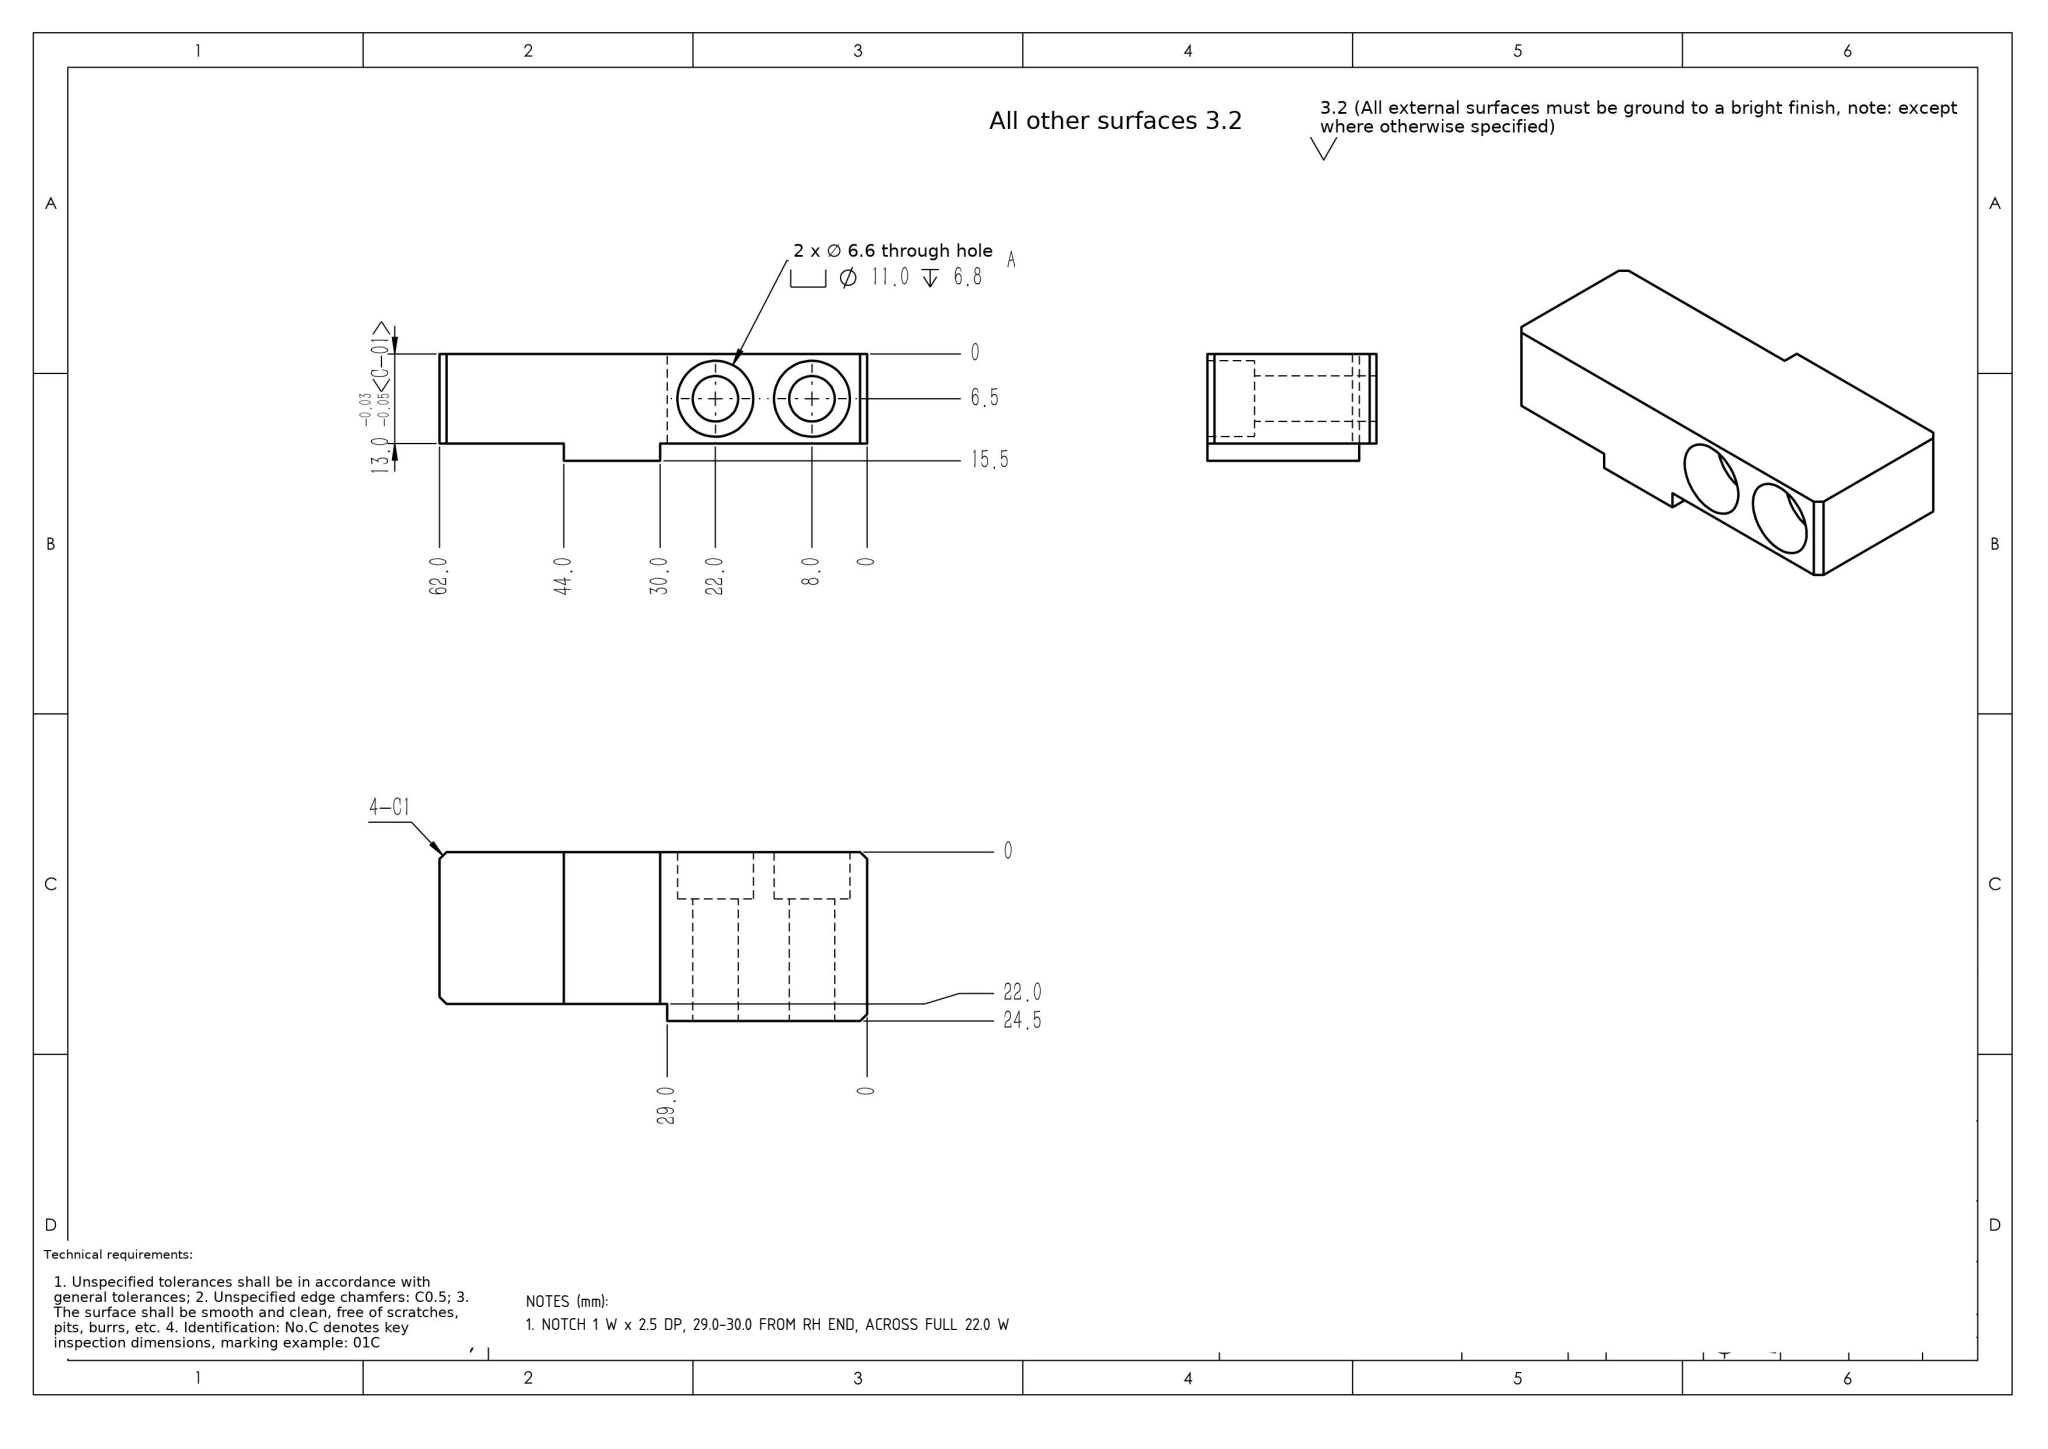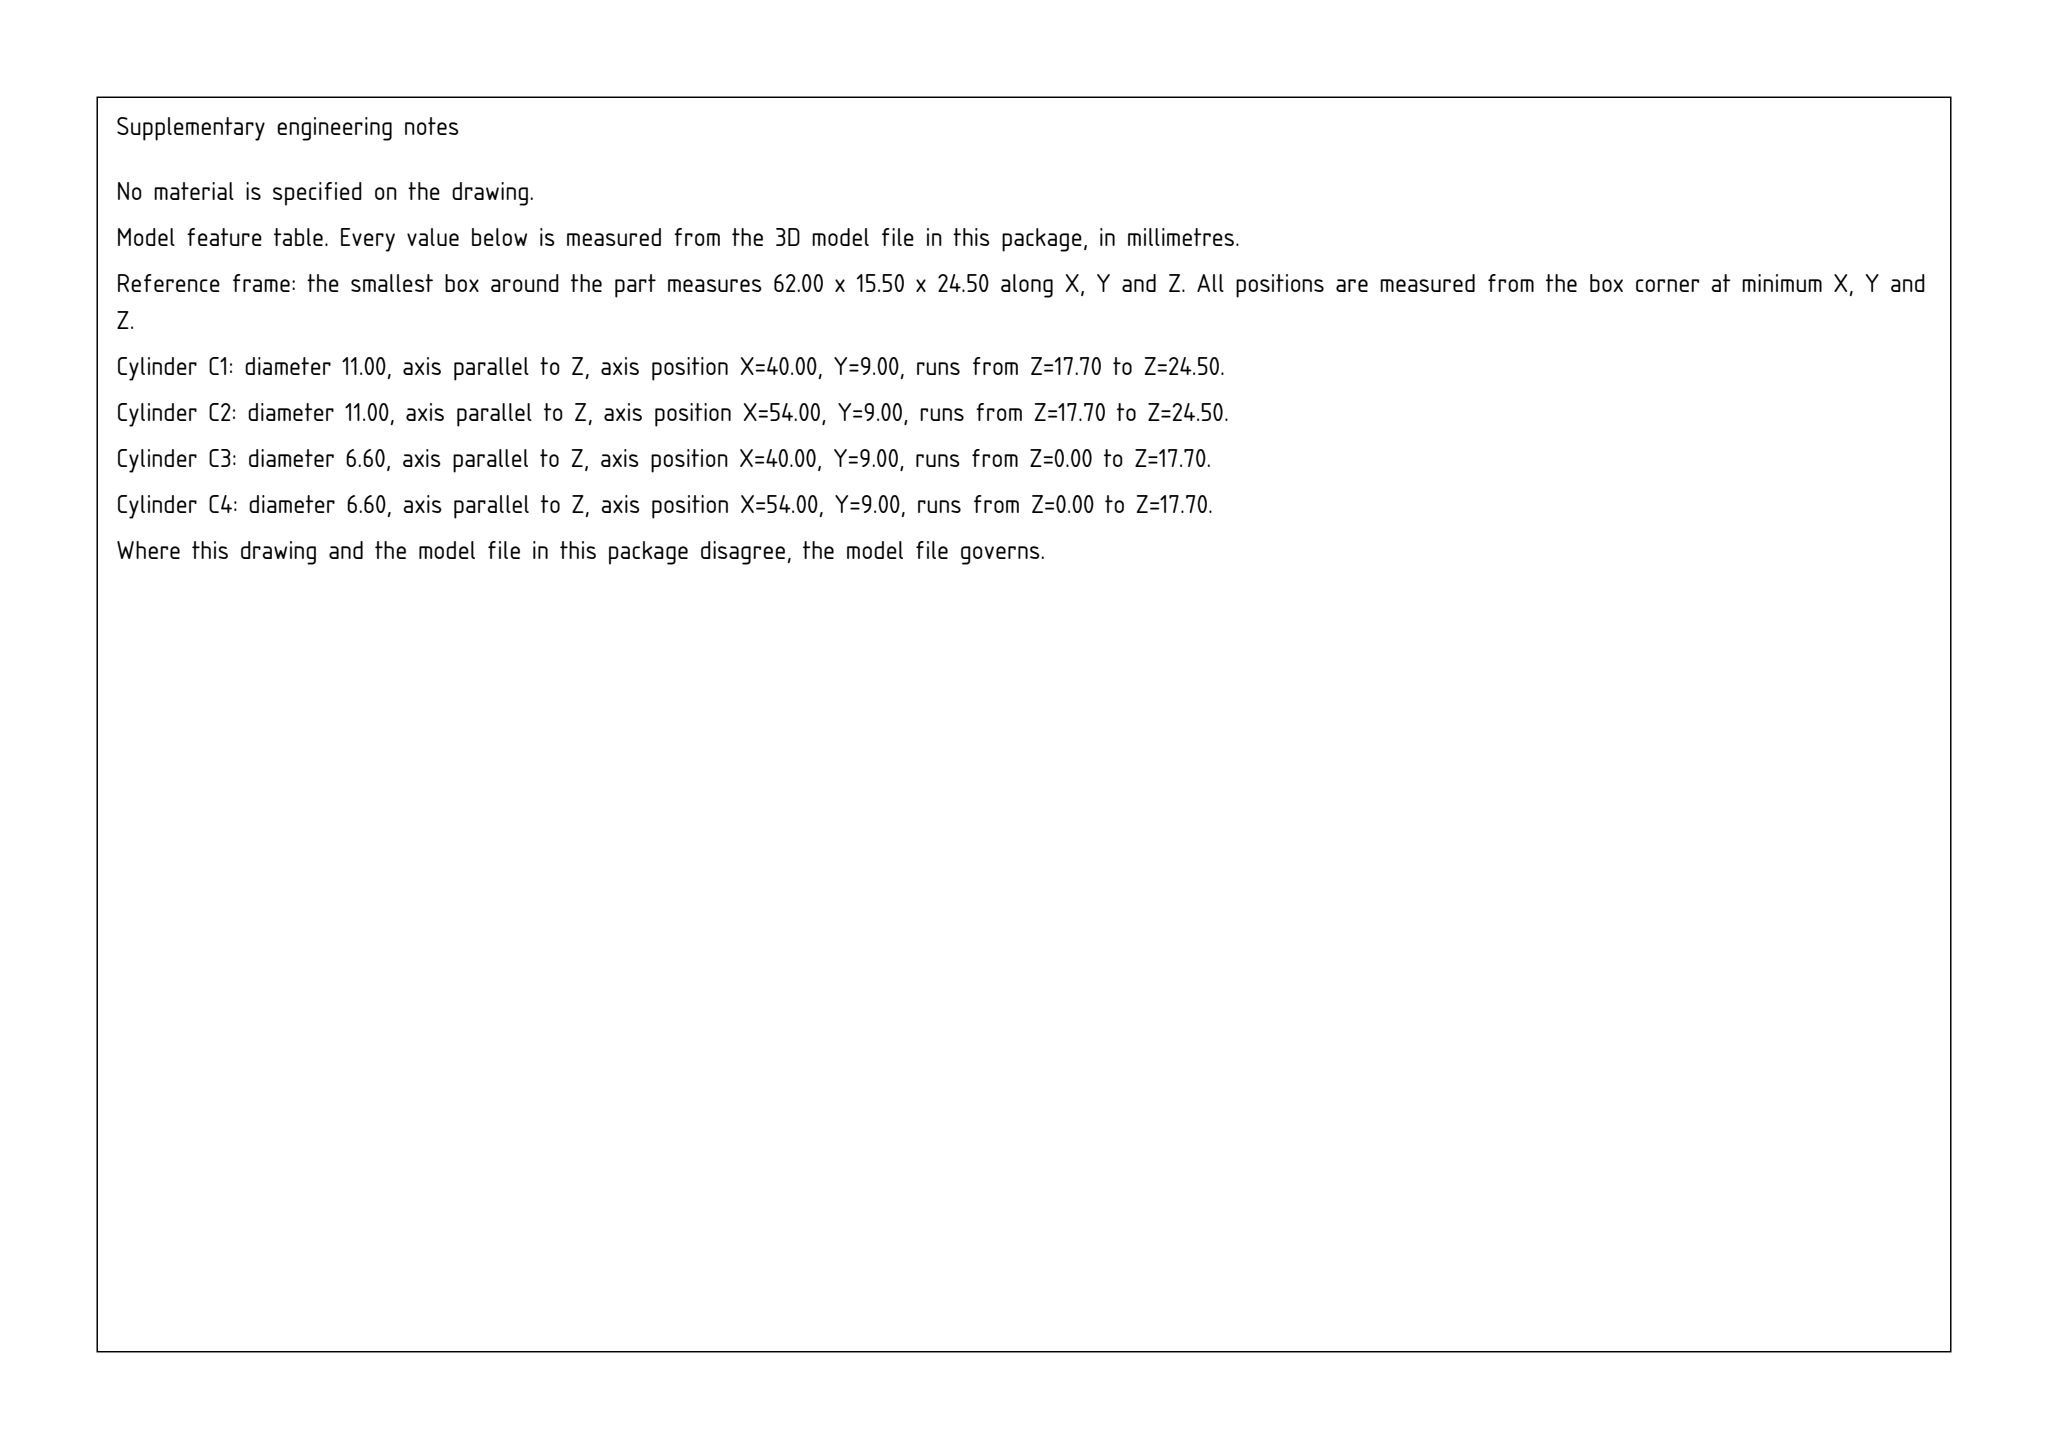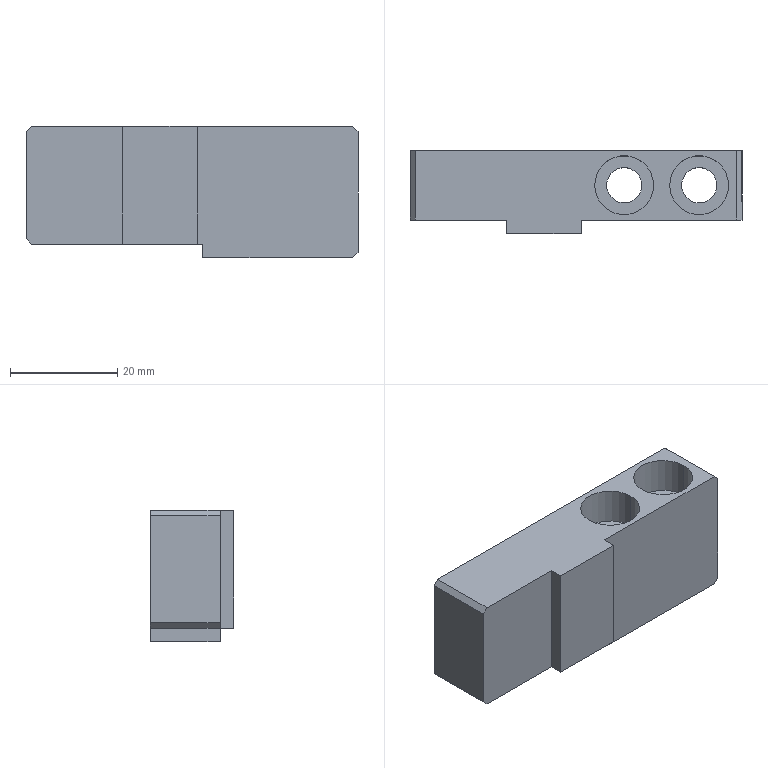Part | SolidWorks | mm | 1 solid | 26 faces | box 62 x 15.5 x 24.5 mm | volume 16915 mm3 | plane 18 | cylinder 8 | commonest cylinder face diameters 11 x4 6.6 x4
Drawing notes:
NOTCH 1 W x 2.5 DP, 29.0-30.0 FROM RH END, ACROSS FULL 22.0 W | from the solid: x-planes 32.0 & 33.0 (=29.0/30.0 from x=62 datum); 2nd y=2.5 face gives 2.5 dp; notch spans z=2.5-24.5 (22.0) as z=0-2.5 ledge ends at x=33
build123d program:
from build123d import *

# Parameters (mm, degrees)
SKETCH1_W                                          = 62
SKETCH1_H                                          = 13
BOSS_EXTRUDE1_DEPTH                                = 24.5
SKETCH2_W                                          = 33
SKETCH2_H                                          = 2.5
CUT_EXTRUDE1_DEPTH                                 = 42.596
HOLE_SIZE_ACCORDING_TO_SLOTTED_PAN_HEA_D           = 6.6
HOLE_SIZE_ACCORDING_TO_SLOTTED_PAN_HEA_CBORE_D     = 11
HOLE_SIZE_ACCORDING_TO_SLOTTED_PAN_HEA_CBORE_DEPTH = 6.8
SKETCH5_W                                          = 32
SKETCH5_H                                          = 2
BOSS_EXTRUDE2_DEPTH                                = 22
SKETCH6_W                                          = 18
SKETCH6_H                                          = 2
CUT_EXTRUDE2_DEPTH                                 = 41.417
CHAMFER1_SIZE                                      = 1
SKETCH7_W                                          = 14
SKETCH7_H                                          = 22
BOSS_EXTRUDE3_DEPTH                                = 0.5


with BuildPart() as part:
    # Sketch1 → Boss-Extrude1 (new body)
    with BuildSketch(Plane.XY):
        Rectangle(SKETCH1_W, SKETCH1_H)
    extrude(amount=BOSS_EXTRUDE1_DEPTH)

    # Sketch2 → Cut-Extrude1 (cut, through all)
    with BuildSketch(Plane(origin=(0, 6.5, 0), x_dir=(1, 0, 0), z_dir=(0, 1, 0))):
        with Locations((-14.5, -1.25)):
            Rectangle(SKETCH2_W, SKETCH2_H)
    extrude(amount=-CUT_EXTRUDE1_DEPTH, mode=Mode.SUBTRACT)

    # Hole Size _According to_ Slotted Pan Hea (through all)
    with Locations(Plane.XY.offset(24.5)):
        with Locations((9, 0), (23, 0)):
            CounterBoreHole(HOLE_SIZE_ACCORDING_TO_SLOTTED_PAN_HEA_D / 2, HOLE_SIZE_ACCORDING_TO_SLOTTED_PAN_HEA_CBORE_D / 2, HOLE_SIZE_ACCORDING_TO_SLOTTED_PAN_HEA_CBORE_DEPTH)

    # Sketch5 → Boss-Extrude2 (add)
    with BuildSketch(Plane.XY.offset(24.5)):
        with Locations((-15, -7.5)):
            Rectangle(SKETCH5_W, SKETCH5_H)
    extrude(amount=-BOSS_EXTRUDE2_DEPTH)

    # Sketch6 → Cut-Extrude2 (cut, through all)
    with BuildSketch(Plane.XY.offset(24.5)):
        with Locations((-22, -7.5)):
            Rectangle(SKETCH6_W, SKETCH6_H)
    extrude(amount=-CUT_EXTRUDE2_DEPTH, mode=Mode.SUBTRACT)

    # Chamfer1
    chamfer1_edges = [part.edges().sort_by_distance(p)[0] for p in [
        (-31, 0, 24.5),
        (31, 0, 24.5),
        (-31, 0, 2.5),
        (31, 0, 0),
    ]]
    chamfer(chamfer1_edges, length=CHAMFER1_SIZE)

    # Sketch7 → Boss-Extrude3 (add)
    with BuildSketch(Plane.XZ.offset(8.5)):
        with Locations((-6, 13.5)):
            Rectangle(SKETCH7_W, SKETCH7_H)
    extrude(amount=BOSS_EXTRUDE3_DEPTH)


solid = part.part
STEP:
#1=CARTESIAN_POINT('',(3.5,0.,17.7));
#2=VERTEX_POINT('',#1);
#3=CARTESIAN_POINT('',(14.5,0.,17.7));
#4=VERTEX_POINT('',#3);
#5=CARTESIAN_POINT('',(9.,0.,17.7));
#6=DIRECTION('',(0.,0.,1.));
#7=DIRECTION('',(1.,0.,0.));
#8=AXIS2_PLACEMENT_3D('',#5,#6,#7);
#9=CIRCLE('',#8,5.5);
#10=EDGE_CURVE('',#2,#4,#9,.T.);
#11=ORIENTED_EDGE('',*,*,#10,.F.);
#12=CARTESIAN_POINT('',(3.5,0.,24.5));
#13=VERTEX_POINT('',#12);
#14=CARTESIAN_POINT('',(3.5,0.,24.5));
#15=DIRECTION('',(0.,0.,1.));
#16=VECTOR('',#15,1000.);
#17=LINE('',#14,#16);
#18=EDGE_CURVE('',#2,#13,#17,.T.);
#19=ORIENTED_EDGE('',*,*,#18,.T.);
#20=CARTESIAN_POINT('',(14.5,0.,24.5));
#21=VERTEX_POINT('',#20);
#22=CARTESIAN_POINT('',(9.,0.,24.5));
#23=DIRECTION('',(0.,0.,1.));
#24=DIRECTION('',(1.,0.,0.));
#25=AXIS2_PLACEMENT_3D('',#22,#23,#24);
#26=CIRCLE('',#25,5.5);
#27=EDGE_CURVE('',#13,#21,#26,.T.);
#28=ORIENTED_EDGE('',*,*,#27,.T.);
#29=CARTESIAN_POINT('',(14.5,0.,24.5));
#30=DIRECTION('',(0.,0.,1.));
#31=VECTOR('',#30,1000.);
#32=LINE('',#29,#31);
#33=EDGE_CURVE('',#4,#21,#32,.T.);
#34=ORIENTED_EDGE('',*,*,#33,.F.);
#35=EDGE_LOOP('',(#11,#19,#28,#34));
#36=FACE_OUTER_BOUND('',#35,.T.);
#37=CARTESIAN_POINT('',(9.,0.,24.5));
#38=DIRECTION('',(0.,0.,1.));
#39=DIRECTION('',(1.,0.,0.));
#40=AXIS2_PLACEMENT_3D('',#37,#38,#39);
#41=CYLINDRICAL_SURFACE('',#40,5.5);
#42=ADVANCED_FACE('',(#36),#41,.F.);
#43=CARTESIAN_POINT('',(5.7,0.,0.));
#44=VERTEX_POINT('',#43);
#45=CARTESIAN_POINT('',(12.3,0.,0.));
#46=VERTEX_POINT('',#45);
#47=CARTESIAN_POINT('',(9.,0.,0.));
#48=DIRECTION('',(0.,0.,1.));
#49=DIRECTION('',(1.,0.,0.));
#50=AXIS2_PLACEMENT_3D('',#47,#48,#49);
#51=CIRCLE('',#50,3.3);
#52=EDGE_CURVE('',#44,#46,#51,.T.);
#53=ORIENTED_EDGE('',*,*,#52,.F.);
#54=CARTESIAN_POINT('',(5.7,0.,17.7));
#55=VERTEX_POINT('',#54);
#56=CARTESIAN_POINT('',(5.7,0.,24.5));
#57=DIRECTION('',(0.,0.,1.));
#58=VECTOR('',#57,1000.);
#59=LINE('',#56,#58);
#60=EDGE_CURVE('',#44,#55,#59,.T.);
#61=ORIENTED_EDGE('',*,*,#60,.T.);
#62=CARTESIAN_POINT('',(12.3,0.,17.7));
#63=VERTEX_POINT('',#62);
#64=CARTESIAN_POINT('',(9.,0.,17.7));
#65=DIRECTION('',(0.,0.,1.));
#66=DIRECTION('',(1.,0.,0.));
#67=AXIS2_PLACEMENT_3D('',#64,#65,#66);
#68=CIRCLE('',#67,3.3);
#69=EDGE_CURVE('',#55,#63,#68,.T.);
#70=ORIENTED_EDGE('',*,*,#69,.T.);
#71=CARTESIAN_POINT('',(12.3,0.,24.5));
#72=DIRECTION('',(0.,0.,1.));
#73=VECTOR('',#72,1000.);
#74=LINE('',#71,#73);
#75=EDGE_CURVE('',#46,#63,#74,.T.);
#76=ORIENTED_EDGE('',*,*,#75,.F.);
#77=EDGE_LOOP('',(#53,#61,#70,#76));
#78=FACE_OUTER_BOUND('',#77,.T.);
#79=CARTESIAN_POINT('',(9.,0.,24.5));
#80=DIRECTION('',(0.,0.,1.));
#81=DIRECTION('',(1.,0.,0.));
#82=AXIS2_PLACEMENT_3D('',#79,#80,#81);
#83=CYLINDRICAL_SURFACE('',#82,3.3);
#84=ADVANCED_FACE('',(#78),#83,.F.);
#85=CARTESIAN_POINT('',(17.5,0.,17.7));
#86=VERTEX_POINT('',#85);
#87=CARTESIAN_POINT('',(28.5,0.,17.7));
#88=VERTEX_POINT('',#87);
#89=CARTESIAN_POINT('',(23.,0.,17.7));
#90=DIRECTION('',(0.,0.,1.));
#91=DIRECTION('',(1.,0.,0.));
#92=AXIS2_PLACEMENT_3D('',#89,#90,#91);
#93=CIRCLE('',#92,5.5);
#94=EDGE_CURVE('',#86,#88,#93,.T.);
#95=ORIENTED_EDGE('',*,*,#94,.F.);
#96=CARTESIAN_POINT('',(17.5,0.,24.5));
#97=VERTEX_POINT('',#96);
#98=CARTESIAN_POINT('',(17.5,0.,24.5));
#99=DIRECTION('',(0.,0.,1.));
#100=VECTOR('',#99,1000.);
#101=LINE('',#98,#100);
#102=EDGE_CURVE('',#86,#97,#101,.T.);
#103=ORIENTED_EDGE('',*,*,#102,.T.);
#104=CARTESIAN_POINT('',(28.5,0.,24.5));
#105=VERTEX_POINT('',#104);
#106=CARTESIAN_POINT('',(23.,0.,24.5));
#107=DIRECTION('',(0.,0.,1.));
#108=DIRECTION('',(1.,0.,0.));
#109=AXIS2_PLACEMENT_3D('',#106,#107,#108);
#110=CIRCLE('',#109,5.5);
#111=EDGE_CURVE('',#97,#105,#110,.T.);
#112=ORIENTED_EDGE('',*,*,#111,.T.);
#113=CARTESIAN_POINT('',(28.5,0.,24.5));
#114=DIRECTION('',(0.,0.,1.));
#115=VECTOR('',#114,1000.);
#116=LINE('',#113,#115);
#117=EDGE_CURVE('',#88,#105,#116,.T.);
#118=ORIENTED_EDGE('',*,*,#117,.F.);
#119=EDGE_LOOP('',(#95,#103,#112,#118));
#120=FACE_OUTER_BOUND('',#119,.T.);
#121=CARTESIAN_POINT('',(23.,0.,24.5));
#122=DIRECTION('',(0.,0.,1.));
#123=DIRECTION('',(1.,0.,0.));
#124=AXIS2_PLACEMENT_3D('',#121,#122,#123);
#125=CYLINDRICAL_SURFACE('',#124,5.5);
#126=ADVANCED_FACE('',(#120),#125,.F.);
#127=CARTESIAN_POINT('',(19.7,0.,0.));
#128=VERTEX_POINT('',#127);
#129=CARTESIAN_POINT('',(26.3,0.,0.));
#130=VERTEX_POINT('',#129);
#131=CARTESIAN_POINT('',(23.,0.,0.));
#132=DIRECTION('',(0.,0.,1.));
#133=DIRECTION('',(1.,0.,0.));
#134=AXIS2_PLACEMENT_3D('',#131,#132,#133);
#135=CIRCLE('',#134,3.3);
#136=EDGE_CURVE('',#128,#130,#135,.T.);
#137=ORIENTED_EDGE('',*,*,#136,.F.);
#138=CARTESIAN_POINT('',(19.7,0.,17.7));
#139=VERTEX_POINT('',#138);
#140=CARTESIAN_POINT('',(19.7,0.,24.5));
#141=DIRECTION('',(0.,0.,1.));
#142=VECTOR('',#141,1000.);
#143=LINE('',#140,#142);
#144=EDGE_CURVE('',#128,#139,#143,.T.);
#145=ORIENTED_EDGE('',*,*,#144,.T.);
#146=CARTESIAN_POINT('',(26.3,0.,17.7));
#147=VERTEX_POINT('',#146);
#148=CARTESIAN_POINT('',(23.,0.,17.7));
#149=DIRECTION('',(0.,0.,1.));
#150=DIRECTION('',(1.,0.,0.));
#151=AXIS2_PLACEMENT_3D('',#148,#149,#150);
#152=CIRCLE('',#151,3.3);
#153=EDGE_CURVE('',#139,#147,#152,.T.);
#154=ORIENTED_EDGE('',*,*,#153,.T.);
#155=CARTESIAN_POINT('',(26.3,0.,24.5));
#156=DIRECTION('',(0.,0.,1.));
#157=VECTOR('',#156,1000.);
#158=LINE('',#155,#157);
#159=EDGE_CURVE('',#130,#147,#158,.T.);
#160=ORIENTED_EDGE('',*,*,#159,.F.);
#161=EDGE_LOOP('',(#137,#145,#154,#160));
#162=FACE_OUTER_BOUND('',#161,.T.);
#163=CARTESIAN_POINT('',(23.,0.,24.5));
#164=DIRECTION('',(0.,0.,1.));
#165=DIRECTION('',(1.,0.,0.));
#166=AXIS2_PLACEMENT_3D('',#163,#164,#165);
#167=CYLINDRICAL_SURFACE('',#166,3.3);
#168=ADVANCED_FACE('',(#162),#167,.F.);
#169=CARTESIAN_POINT('',(2.,-6.5,0.));
#170=VERTEX_POINT('',#169);
#171=CARTESIAN_POINT('',(30.,-6.5,-0.));
#172=VERTEX_POINT('',#171);
#173=CARTESIAN_POINT('',(-31.,-6.5,0.));
#174=DIRECTION('',(1.,0.,0.));
#175=VECTOR('',#174,1000.);
#176=LINE('',#173,#175);
#177=EDGE_CURVE('',#170,#172,#176,.T.);
#178=ORIENTED_EDGE('',*,*,#177,.T.);
#179=CARTESIAN_POINT('',(31.,-6.5,1.));
#180=VERTEX_POINT('',#179);
#181=CARTESIAN_POINT('',(31.,-6.5,1.));
#182=DIRECTION('',(0.7071,0.,0.7071));
#183=VECTOR('',#182,1000.);
#184=LINE('',#181,#183);
#185=EDGE_CURVE('',#172,#180,#184,.T.);
#186=ORIENTED_EDGE('',*,*,#185,.T.);
#187=CARTESIAN_POINT('',(31.,-6.5,23.5));
#188=VERTEX_POINT('',#187);
#189=CARTESIAN_POINT('',(31.,-6.5,24.5));
#190=DIRECTION('',(0.,0.,-1.));
#191=VECTOR('',#190,1000.);
#192=LINE('',#189,#191);
#193=EDGE_CURVE('',#188,#180,#192,.T.);
#194=ORIENTED_EDGE('',*,*,#193,.F.);
#195=CARTESIAN_POINT('',(30.,-6.5,24.5));
#196=VERTEX_POINT('',#195);
#197=CARTESIAN_POINT('',(30.,-6.5,24.5));
#198=DIRECTION('',(-0.7071,0.,0.7071));
#199=VECTOR('',#198,1000.);
#200=LINE('',#197,#199);
#201=EDGE_CURVE('',#188,#196,#200,.T.);
#202=ORIENTED_EDGE('',*,*,#201,.T.);
#203=CARTESIAN_POINT('',(1.,-6.5,24.5));
#204=VERTEX_POINT('',#203);
#205=CARTESIAN_POINT('',(-31.,-6.5,24.5));
#206=DIRECTION('',(1.,0.,0.));
#207=VECTOR('',#206,1000.);
#208=LINE('',#205,#207);
#209=EDGE_CURVE('',#204,#196,#208,.T.);
#210=ORIENTED_EDGE('',*,*,#209,.F.);
#211=CARTESIAN_POINT('',(1.,-6.5,2.5));
#212=VERTEX_POINT('',#211);
#213=CARTESIAN_POINT('',(1.,-6.5,-29.562));
#214=DIRECTION('',(0.,0.,1.));
#215=VECTOR('',#214,1000.);
#216=LINE('',#213,#215);
#217=EDGE_CURVE('',#212,#204,#216,.T.);
#218=ORIENTED_EDGE('',*,*,#217,.F.);
#219=CARTESIAN_POINT('',(2.,-6.5,2.5));
#220=VERTEX_POINT('',#219);
#221=CARTESIAN_POINT('',(-31.,-6.5,2.5));
#222=DIRECTION('',(1.,0.,0.));
#223=VECTOR('',#222,1000.);
#224=LINE('',#221,#223);
#225=EDGE_CURVE('',#212,#220,#224,.T.);
#226=ORIENTED_EDGE('',*,*,#225,.T.);
#227=CARTESIAN_POINT('',(2.,-6.5,0.));
#228=DIRECTION('',(-0.,0.,-1.));
#229=VECTOR('',#228,1000.);
#230=LINE('',#227,#229);
#231=EDGE_CURVE('',#220,#170,#230,.T.);
#232=ORIENTED_EDGE('',*,*,#231,.T.);
#233=EDGE_LOOP('',(#178,#186,#194,#202,#210,#218,#226,#232));
#234=FACE_OUTER_BOUND('',#233,.T.);
#235=CARTESIAN_POINT('',(-31.,-6.5,24.5));
#236=DIRECTION('',(0.,1.,0.));
#237=DIRECTION('',(0.,0.,1.));
#238=AXIS2_PLACEMENT_3D('',#235,#236,#237);
#239=PLANE('',#238);
#240=ADVANCED_FACE('',(#234),#239,.F.);
#241=ORIENTED_EDGE('',*,*,#193,.T.);
#242=CARTESIAN_POINT('',(31.,6.5,1.));
#243=VERTEX_POINT('',#242);
#244=CARTESIAN_POINT('',(31.,6.5,1.));
#245=DIRECTION('',(-0.,1.,0.));
#246=VECTOR('',#245,1000.);
#247=LINE('',#244,#246);
#248=EDGE_CURVE('',#180,#243,#247,.T.);
#249=ORIENTED_EDGE('',*,*,#248,.T.);
#250=CARTESIAN_POINT('',(31.,6.5,23.5));
#251=VERTEX_POINT('',#250);
#252=CARTESIAN_POINT('',(31.,6.5,24.5));
#253=DIRECTION('',(0.,0.,-1.));
#254=VECTOR('',#253,1000.);
#255=LINE('',#252,#254);
#256=EDGE_CURVE('',#251,#243,#255,.T.);
#257=ORIENTED_EDGE('',*,*,#256,.F.);
#258=CARTESIAN_POINT('',(31.,-6.5,23.5));
#259=DIRECTION('',(0.,-1.,0.));
#260=VECTOR('',#259,1000.);
#261=LINE('',#258,#260);
#262=EDGE_CURVE('',#251,#188,#261,.T.);
#263=ORIENTED_EDGE('',*,*,#262,.T.);
#264=EDGE_LOOP('',(#241,#249,#257,#263));
#265=FACE_OUTER_BOUND('',#264,.T.);
#266=CARTESIAN_POINT('',(31.,6.5,24.5));
#267=DIRECTION('',(-1.,-0.,0.));
#268=DIRECTION('',(0.,-1.,0.));
#269=AXIS2_PLACEMENT_3D('',#266,#267,#268);
#270=PLANE('',#269);
#271=ADVANCED_FACE('',(#265),#270,.F.);
#272=ORIENTED_EDGE('',*,*,#256,.T.);
#273=CARTESIAN_POINT('',(30.,6.5,0.));
#274=VERTEX_POINT('',#273);
#275=CARTESIAN_POINT('',(31.,6.5,1.));
#276=DIRECTION('',(-0.7071,0.,-0.7071));
#277=VECTOR('',#276,1000.);
#278=LINE('',#275,#277);
#279=EDGE_CURVE('',#243,#274,#278,.T.);
#280=ORIENTED_EDGE('',*,*,#279,.T.);
#281=CARTESIAN_POINT('',(2.,6.5,0.));
#282=VERTEX_POINT('',#281);
#283=CARTESIAN_POINT('',(-31.,6.5,0.));
#284=DIRECTION('',(-1.,0.,0.));
#285=VECTOR('',#284,1000.);
#286=LINE('',#283,#285);
#287=EDGE_CURVE('',#274,#282,#286,.T.);
#288=ORIENTED_EDGE('',*,*,#287,.T.);
#289=CARTESIAN_POINT('',(2.,6.5,2.5));
#290=VERTEX_POINT('',#289);
#291=CARTESIAN_POINT('',(2.,6.5,0.));
#292=DIRECTION('',(-0.,0.,-1.));
#293=VECTOR('',#292,1000.);
#294=LINE('',#291,#293);
#295=EDGE_CURVE('',#290,#282,#294,.T.);
#296=ORIENTED_EDGE('',*,*,#295,.F.);
#297=CARTESIAN_POINT('',(-30.,6.5,2.5));
#298=VERTEX_POINT('',#297);
#299=CARTESIAN_POINT('',(-31.,6.5,2.5));
#300=DIRECTION('',(1.,0.,0.));
#301=VECTOR('',#300,1000.);
#302=LINE('',#299,#301);
#303=EDGE_CURVE('',#298,#290,#302,.T.);
#304=ORIENTED_EDGE('',*,*,#303,.F.);
#305=CARTESIAN_POINT('',(-31.,6.5,3.5));
#306=VERTEX_POINT('',#305);
#307=CARTESIAN_POINT('',(-30.,6.5,2.5));
#308=DIRECTION('',(-0.7071,0.,0.7071));
#309=VECTOR('',#308,1000.);
#310=LINE('',#307,#309);
#311=EDGE_CURVE('',#298,#306,#310,.T.);
#312=ORIENTED_EDGE('',*,*,#311,.T.);
#313=CARTESIAN_POINT('',(-31.,6.5,23.5));
#314=VERTEX_POINT('',#313);
#315=CARTESIAN_POINT('',(-31.,6.5,24.5));
#316=DIRECTION('',(0.,0.,-1.));
#317=VECTOR('',#316,1000.);
#318=LINE('',#315,#317);
#319=EDGE_CURVE('',#314,#306,#318,.T.);
#320=ORIENTED_EDGE('',*,*,#319,.F.);
#321=CARTESIAN_POINT('',(-30.,6.5,24.5));
#322=VERTEX_POINT('',#321);
#323=CARTESIAN_POINT('',(-30.,6.5,24.5));
#324=DIRECTION('',(0.7071,0.,0.7071));
#325=VECTOR('',#324,1000.);
#326=LINE('',#323,#325);
#327=EDGE_CURVE('',#314,#322,#326,.T.);
#328=ORIENTED_EDGE('',*,*,#327,.T.);
#329=CARTESIAN_POINT('',(30.,6.5,24.5));
#330=VERTEX_POINT('',#329);
#331=CARTESIAN_POINT('',(-31.,6.5,24.5));
#332=DIRECTION('',(-1.,0.,0.));
#333=VECTOR('',#332,1000.);
#334=LINE('',#331,#333);
#335=EDGE_CURVE('',#330,#322,#334,.T.);
#336=ORIENTED_EDGE('',*,*,#335,.F.);
#337=CARTESIAN_POINT('',(30.,6.5,24.5));
#338=DIRECTION('',(0.7071,0.,-0.7071));
#339=VECTOR('',#338,1000.);
#340=LINE('',#337,#339);
#341=EDGE_CURVE('',#330,#251,#340,.T.);
#342=ORIENTED_EDGE('',*,*,#341,.T.);
#343=EDGE_LOOP('',(#272,#280,#288,#296,#304,#312,#320,#328,#336,#342));
#344=FACE_OUTER_BOUND('',#343,.T.);
#345=CARTESIAN_POINT('',(-31.,6.5,24.5));
#346=DIRECTION('',(0.,-1.,0.));
#347=DIRECTION('',(0.,0.,-1.));
#348=AXIS2_PLACEMENT_3D('',#345,#346,#347);
#349=PLANE('',#348);
#350=ADVANCED_FACE('',(#344),#349,.F.);
#351=ORIENTED_EDGE('',*,*,#319,.T.);
#352=CARTESIAN_POINT('',(-31.,-6.5,3.5));
#353=VERTEX_POINT('',#352);
#354=CARTESIAN_POINT('',(-31.,6.5,3.5));
#355=DIRECTION('',(0.,-1.,0.));
#356=VECTOR('',#355,1000.);
#357=LINE('',#354,#356);
#358=EDGE_CURVE('',#306,#353,#357,.T.);
#359=ORIENTED_EDGE('',*,*,#358,.T.);
#360=CARTESIAN_POINT('',(-31.,-6.5,23.5));
#361=VERTEX_POINT('',#360);
#362=CARTESIAN_POINT('',(-31.,-6.5,0.));
#363=DIRECTION('',(0.,0.,1.));
#364=VECTOR('',#363,1000.);
#365=LINE('',#362,#364);
#366=EDGE_CURVE('',#353,#361,#365,.T.);
#367=ORIENTED_EDGE('',*,*,#366,.T.);
#368=CARTESIAN_POINT('',(-31.,6.5,23.5));
#369=DIRECTION('',(-0.,1.,0.));
#370=VECTOR('',#369,1000.);
#371=LINE('',#368,#370);
#372=EDGE_CURVE('',#361,#314,#371,.T.);
#373=ORIENTED_EDGE('',*,*,#372,.T.);
#374=EDGE_LOOP('',(#351,#359,#367,#373));
#375=FACE_OUTER_BOUND('',#374,.T.);
#376=CARTESIAN_POINT('',(-31.,6.5,24.5));
#377=DIRECTION('',(1.,0.,0.));
#378=DIRECTION('',(-0.,1.,0.));
#379=AXIS2_PLACEMENT_3D('',#376,#377,#378);
#380=PLANE('',#379);
#381=ADVANCED_FACE('',(#375),#380,.F.);
#382=ORIENTED_EDGE('',*,*,#209,.T.);
#383=CARTESIAN_POINT('',(30.,6.5,24.5));
#384=DIRECTION('',(-0.,1.,0.));
#385=VECTOR('',#384,1000.);
#386=LINE('',#383,#385);
#387=EDGE_CURVE('',#196,#330,#386,.T.);
#388=ORIENTED_EDGE('',*,*,#387,.T.);
#389=ORIENTED_EDGE('',*,*,#335,.T.);
#390=CARTESIAN_POINT('',(-30.,-6.5,24.5));
#391=VERTEX_POINT('',#390);
#392=CARTESIAN_POINT('',(-30.,-6.5,24.5));
#393=DIRECTION('',(0.,-1.,0.));
#394=VECTOR('',#393,1000.);
#395=LINE('',#392,#394);
#396=EDGE_CURVE('',#322,#391,#395,.T.);
#397=ORIENTED_EDGE('',*,*,#396,.T.);
#398=CARTESIAN_POINT('',(-13.,-6.5,24.5));
#399=VERTEX_POINT('',#398);
#400=CARTESIAN_POINT('',(-31.,-6.5,24.5));
#401=DIRECTION('',(-1.,0.,0.));
#402=VECTOR('',#401,1000.);
#403=LINE('',#400,#402);
#404=EDGE_CURVE('',#399,#391,#403,.T.);
#405=ORIENTED_EDGE('',*,*,#404,.F.);
#406=CARTESIAN_POINT('',(-13.,-9.,24.5));
#407=VERTEX_POINT('',#406);
#408=CARTESIAN_POINT('',(-13.,-8.5,24.5));
#409=DIRECTION('',(0.,1.,0.));
#410=VECTOR('',#409,1000.);
#411=LINE('',#408,#410);
#412=EDGE_CURVE('',#407,#399,#411,.T.);
#413=ORIENTED_EDGE('',*,*,#412,.F.);
#414=CARTESIAN_POINT('',(1.,-9.,24.5));
#415=VERTEX_POINT('',#414);
#416=CARTESIAN_POINT('',(-13.,-9.,24.5));
#417=DIRECTION('',(-1.,0.,0.));
#418=VECTOR('',#417,1000.);
#419=LINE('',#416,#418);
#420=EDGE_CURVE('',#415,#407,#419,.T.);
#421=ORIENTED_EDGE('',*,*,#420,.F.);
#422=CARTESIAN_POINT('',(1.,-6.5,24.5));
#423=DIRECTION('',(-0.,1.,0.));
#424=VECTOR('',#423,1000.);
#425=LINE('',#422,#424);
#426=EDGE_CURVE('',#415,#204,#425,.T.);
#427=ORIENTED_EDGE('',*,*,#426,.T.);
#428=EDGE_LOOP('',(#382,#388,#389,#397,#405,#413,#421,#427));
#429=FACE_OUTER_BOUND('',#428,.T.);
#430=CARTESIAN_POINT('',(9.,0.,24.5));
#431=DIRECTION('',(0.,0.,1.));
#432=DIRECTION('',(1.,0.,0.));
#433=AXIS2_PLACEMENT_3D('',#430,#431,#432);
#434=CIRCLE('',#433,5.5);
#435=EDGE_CURVE('',#21,#13,#434,.T.);
#436=ORIENTED_EDGE('',*,*,#435,.F.);
#437=ORIENTED_EDGE('',*,*,#27,.F.);
#438=EDGE_LOOP('',(#436,#437));
#439=FACE_BOUND('',#438,.T.);
#440=CARTESIAN_POINT('',(23.,0.,24.5));
#441=DIRECTION('',(0.,0.,1.));
#442=DIRECTION('',(1.,0.,0.));
#443=AXIS2_PLACEMENT_3D('',#440,#441,#442);
#444=CIRCLE('',#443,5.5);
#445=EDGE_CURVE('',#105,#97,#444,.T.);
#446=ORIENTED_EDGE('',*,*,#445,.F.);
#447=ORIENTED_EDGE('',*,*,#111,.F.);
#448=EDGE_LOOP('',(#446,#447));
#449=FACE_BOUND('',#448,.T.);
#450=CARTESIAN_POINT('',(0.,0.,24.5));
#451=DIRECTION('',(0.,0.,1.));
#452=DIRECTION('',(1.,0.,0.));
#453=AXIS2_PLACEMENT_3D('',#450,#451,#452);
#454=PLANE('',#453);
#455=ADVANCED_FACE('',(#429,#439,#449),#454,.T.);
#456=CARTESIAN_POINT('',(9.,0.,0.));
#457=DIRECTION('',(0.,0.,1.));
#458=DIRECTION('',(1.,0.,0.));
#459=AXIS2_PLACEMENT_3D('',#456,#457,#458);
#460=CIRCLE('',#459,3.3);
#461=EDGE_CURVE('',#46,#44,#460,.T.);
#462=ORIENTED_EDGE('',*,*,#461,.T.);
#463=ORIENTED_EDGE('',*,*,#52,.T.);
#464=EDGE_LOOP('',(#462,#463));
#465=FACE_BOUND('',#464,.T.);
#466=CARTESIAN_POINT('',(23.,0.,0.));
#467=DIRECTION('',(0.,0.,1.));
#468=DIRECTION('',(1.,0.,0.));
#469=AXIS2_PLACEMENT_3D('',#466,#467,#468);
#470=CIRCLE('',#469,3.3);
#471=EDGE_CURVE('',#130,#128,#470,.T.);
#472=ORIENTED_EDGE('',*,*,#471,.T.);
#473=ORIENTED_EDGE('',*,*,#136,.T.);
#474=EDGE_LOOP('',(#472,#473));
#475=FACE_BOUND('',#474,.T.);
#476=ORIENTED_EDGE('',*,*,#287,.F.);
#477=CARTESIAN_POINT('',(30.,0.,0.));
#478=DIRECTION('',(0.,-1.,0.));
#479=VECTOR('',#478,1000.);
#480=LINE('',#477,#479);
#481=EDGE_CURVE('',#274,#172,#480,.T.);
#482=ORIENTED_EDGE('',*,*,#481,.T.);
#483=ORIENTED_EDGE('',*,*,#177,.F.);
#484=CARTESIAN_POINT('',(2.,-6.5,0.));
#485=DIRECTION('',(0.,1.,0.));
#486=VECTOR('',#485,1000.);
#487=LINE('',#484,#486);
#488=EDGE_CURVE('',#170,#282,#487,.T.);
#489=ORIENTED_EDGE('',*,*,#488,.T.);
#490=EDGE_LOOP('',(#476,#482,#483,#489));
#491=FACE_OUTER_BOUND('',#490,.T.);
#492=CARTESIAN_POINT('',(0.,0.,0.));
#493=DIRECTION('',(0.,0.,1.));
#494=DIRECTION('',(1.,0.,0.));
#495=AXIS2_PLACEMENT_3D('',#492,#493,#494);
#496=PLANE('',#495);
#497=ADVANCED_FACE('',(#465,#475,#491),#496,.F.);
#498=ORIENTED_EDGE('',*,*,#295,.T.);
#499=ORIENTED_EDGE('',*,*,#488,.F.);
#500=ORIENTED_EDGE('',*,*,#231,.F.);
#501=CARTESIAN_POINT('',(2.,-6.5,2.5));
#502=DIRECTION('',(0.,1.,0.));
#503=VECTOR('',#502,1000.);
#504=LINE('',#501,#503);
#505=EDGE_CURVE('',#220,#290,#504,.T.);
#506=ORIENTED_EDGE('',*,*,#505,.T.);
#507=EDGE_LOOP('',(#498,#499,#500,#506));
#508=FACE_OUTER_BOUND('',#507,.T.);
#509=CARTESIAN_POINT('',(2.,-6.5,0.));
#510=DIRECTION('',(1.,0.,-0.));
#511=DIRECTION('',(-0.,0.,-1.));
#512=AXIS2_PLACEMENT_3D('',#509,#510,#511);
#513=PLANE('',#512);
#514=ADVANCED_FACE('',(#508),#513,.F.);
#515=CARTESIAN_POINT('',(-13.,-6.5,2.5));
#516=VERTEX_POINT('',#515);
#517=CARTESIAN_POINT('',(-30.,-6.5,2.5));
#518=VERTEX_POINT('',#517);
#519=CARTESIAN_POINT('',(-31.,-6.5,2.5));
#520=DIRECTION('',(-1.,0.,0.));
#521=VECTOR('',#520,1000.);
#522=LINE('',#519,#521);
#523=EDGE_CURVE('',#516,#518,#522,.T.);
#524=ORIENTED_EDGE('',*,*,#523,.T.);
#525=CARTESIAN_POINT('',(-30.,-6.5,2.5));
#526=DIRECTION('',(-0.,1.,0.));
#527=VECTOR('',#526,1000.);
#528=LINE('',#525,#527);
#529=EDGE_CURVE('',#518,#298,#528,.T.);
#530=ORIENTED_EDGE('',*,*,#529,.T.);
#531=ORIENTED_EDGE('',*,*,#303,.T.);
#532=ORIENTED_EDGE('',*,*,#505,.F.);
#533=ORIENTED_EDGE('',*,*,#225,.F.);
#534=CARTESIAN_POINT('',(1.,-9.,2.5));
#535=VERTEX_POINT('',#534);
#536=CARTESIAN_POINT('',(1.,-6.5,2.5));
#537=DIRECTION('',(0.,-1.,0.));
#538=VECTOR('',#537,1000.);
#539=LINE('',#536,#538);
#540=EDGE_CURVE('',#212,#535,#539,.T.);
#541=ORIENTED_EDGE('',*,*,#540,.T.);
#542=CARTESIAN_POINT('',(-13.,-9.,2.5));
#543=VERTEX_POINT('',#542);
#544=CARTESIAN_POINT('',(-13.,-9.,2.5));
#545=DIRECTION('',(1.,0.,0.));
#546=VECTOR('',#545,1000.);
#547=LINE('',#544,#546);
#548=EDGE_CURVE('',#543,#535,#547,.T.);
#549=ORIENTED_EDGE('',*,*,#548,.F.);
#550=CARTESIAN_POINT('',(-13.,-6.5,2.5));
#551=DIRECTION('',(0.,1.,0.));
#552=VECTOR('',#551,1000.);
#553=LINE('',#550,#552);
#554=EDGE_CURVE('',#543,#516,#553,.T.);
#555=ORIENTED_EDGE('',*,*,#554,.T.);
#556=EDGE_LOOP('',(#524,#530,#531,#532,#533,#541,#549,#555));
#557=FACE_OUTER_BOUND('',#556,.T.);
#558=CARTESIAN_POINT('',(-31.,-6.5,2.5));
#559=DIRECTION('',(0.,0.,1.));
#560=DIRECTION('',(1.,0.,0.));
#561=AXIS2_PLACEMENT_3D('',#558,#559,#560);
#562=PLANE('',#561);
#563=ADVANCED_FACE('',(#557),#562,.F.);
#564=ORIENTED_EDGE('',*,*,#144,.F.);
#565=ORIENTED_EDGE('',*,*,#471,.F.);
#566=ORIENTED_EDGE('',*,*,#159,.T.);
#567=CARTESIAN_POINT('',(23.,0.,17.7));
#568=DIRECTION('',(0.,0.,1.));
#569=DIRECTION('',(1.,0.,0.));
#570=AXIS2_PLACEMENT_3D('',#567,#568,#569);
#571=CIRCLE('',#570,3.3);
#572=EDGE_CURVE('',#147,#139,#571,.T.);
#573=ORIENTED_EDGE('',*,*,#572,.T.);
#574=EDGE_LOOP('',(#564,#565,#566,#573));
#575=FACE_OUTER_BOUND('',#574,.T.);
#576=CARTESIAN_POINT('',(23.,0.,24.5));
#577=DIRECTION('',(0.,0.,1.));
#578=DIRECTION('',(1.,0.,0.));
#579=AXIS2_PLACEMENT_3D('',#576,#577,#578);
#580=CYLINDRICAL_SURFACE('',#579,3.3);
#581=ADVANCED_FACE('',(#575),#580,.F.);
#582=ORIENTED_EDGE('',*,*,#572,.F.);
#583=ORIENTED_EDGE('',*,*,#153,.F.);
#584=EDGE_LOOP('',(#582,#583));
#585=FACE_BOUND('',#584,.T.);
#586=CARTESIAN_POINT('',(23.,0.,17.7));
#587=DIRECTION('',(0.,0.,1.));
#588=DIRECTION('',(1.,0.,0.));
#589=AXIS2_PLACEMENT_3D('',#586,#587,#588);
#590=CIRCLE('',#589,5.5);
#591=EDGE_CURVE('',#88,#86,#590,.T.);
#592=ORIENTED_EDGE('',*,*,#591,.T.);
#593=ORIENTED_EDGE('',*,*,#94,.T.);
#594=EDGE_LOOP('',(#592,#593));
#595=FACE_OUTER_BOUND('',#594,.T.);
#596=CARTESIAN_POINT('',(26.3,0.,17.7));
#597=DIRECTION('',(0.,0.,-1.));
#598=DIRECTION('',(-1.,0.,0.));
#599=AXIS2_PLACEMENT_3D('',#596,#597,#598);
#600=PLANE('',#599);
#601=ADVANCED_FACE('',(#585,#595),#600,.F.);
#602=ORIENTED_EDGE('',*,*,#102,.F.);
#603=ORIENTED_EDGE('',*,*,#591,.F.);
#604=ORIENTED_EDGE('',*,*,#117,.T.);
#605=ORIENTED_EDGE('',*,*,#445,.T.);
#606=EDGE_LOOP('',(#602,#603,#604,#605));
#607=FACE_OUTER_BOUND('',#606,.T.);
#608=CARTESIAN_POINT('',(23.,0.,24.5));
#609=DIRECTION('',(0.,0.,1.));
#610=DIRECTION('',(1.,0.,0.));
#611=AXIS2_PLACEMENT_3D('',#608,#609,#610);
#612=CYLINDRICAL_SURFACE('',#611,5.5);
#613=ADVANCED_FACE('',(#607),#612,.F.);
#614=ORIENTED_EDGE('',*,*,#60,.F.);
#615=ORIENTED_EDGE('',*,*,#461,.F.);
#616=ORIENTED_EDGE('',*,*,#75,.T.);
#617=CARTESIAN_POINT('',(9.,0.,17.7));
#618=DIRECTION('',(0.,0.,1.));
#619=DIRECTION('',(1.,0.,0.));
#620=AXIS2_PLACEMENT_3D('',#617,#618,#619);
#621=CIRCLE('',#620,3.3);
#622=EDGE_CURVE('',#63,#55,#621,.T.);
#623=ORIENTED_EDGE('',*,*,#622,.T.);
#624=EDGE_LOOP('',(#614,#615,#616,#623));
#625=FACE_OUTER_BOUND('',#624,.T.);
#626=CARTESIAN_POINT('',(9.,0.,24.5));
#627=DIRECTION('',(0.,0.,1.));
#628=DIRECTION('',(1.,0.,0.));
#629=AXIS2_PLACEMENT_3D('',#626,#627,#628);
#630=CYLINDRICAL_SURFACE('',#629,3.3);
#631=ADVANCED_FACE('',(#625),#630,.F.);
#632=ORIENTED_EDGE('',*,*,#622,.F.);
#633=ORIENTED_EDGE('',*,*,#69,.F.);
#634=EDGE_LOOP('',(#632,#633));
#635=FACE_BOUND('',#634,.T.);
#636=CARTESIAN_POINT('',(9.,0.,17.7));
#637=DIRECTION('',(0.,0.,1.));
#638=DIRECTION('',(1.,0.,0.));
#639=AXIS2_PLACEMENT_3D('',#636,#637,#638);
#640=CIRCLE('',#639,5.5);
#641=EDGE_CURVE('',#4,#2,#640,.T.);
#642=ORIENTED_EDGE('',*,*,#641,.T.);
#643=ORIENTED_EDGE('',*,*,#10,.T.);
#644=EDGE_LOOP('',(#642,#643));
#645=FACE_OUTER_BOUND('',#644,.T.);
#646=CARTESIAN_POINT('',(12.3,0.,17.7));
#647=DIRECTION('',(0.,0.,-1.));
#648=DIRECTION('',(-1.,0.,0.));
#649=AXIS2_PLACEMENT_3D('',#646,#647,#648);
#650=PLANE('',#649);
#651=ADVANCED_FACE('',(#635,#645),#650,.F.);
#652=ORIENTED_EDGE('',*,*,#18,.F.);
#653=ORIENTED_EDGE('',*,*,#641,.F.);
#654=ORIENTED_EDGE('',*,*,#33,.T.);
#655=ORIENTED_EDGE('',*,*,#435,.T.);
#656=EDGE_LOOP('',(#652,#653,#654,#655));
#657=FACE_OUTER_BOUND('',#656,.T.);
#658=CARTESIAN_POINT('',(9.,0.,24.5));
#659=DIRECTION('',(0.,0.,1.));
#660=DIRECTION('',(1.,0.,0.));
#661=AXIS2_PLACEMENT_3D('',#658,#659,#660);
#662=CYLINDRICAL_SURFACE('',#661,5.5);
#663=ADVANCED_FACE('',(#657),#662,.F.);
#664=ORIENTED_EDGE('',*,*,#540,.F.);
#665=ORIENTED_EDGE('',*,*,#217,.T.);
#666=ORIENTED_EDGE('',*,*,#426,.F.);
#667=CARTESIAN_POINT('',(1.,-9.,24.5));
#668=DIRECTION('',(0.,0.,1.));
#669=VECTOR('',#668,1000.);
#670=LINE('',#667,#669);
#671=EDGE_CURVE('',#535,#415,#670,.T.);
#672=ORIENTED_EDGE('',*,*,#671,.F.);
#673=EDGE_LOOP('',(#664,#665,#666,#672));
#674=FACE_OUTER_BOUND('',#673,.T.);
#675=CARTESIAN_POINT('',(1.,-6.5,-29.562));
#676=DIRECTION('',(1.,0.,0.));
#677=DIRECTION('',(-0.,1.,0.));
#678=AXIS2_PLACEMENT_3D('',#675,#676,#677);
#679=PLANE('',#678);
#680=ADVANCED_FACE('',(#674),#679,.T.);
#681=ORIENTED_EDGE('',*,*,#366,.F.);
#682=CARTESIAN_POINT('',(-30.,-6.5,2.5));
#683=DIRECTION('',(0.7071,0.,-0.7071));
#684=VECTOR('',#683,1000.);
#685=LINE('',#682,#684);
#686=EDGE_CURVE('',#353,#518,#685,.T.);
#687=ORIENTED_EDGE('',*,*,#686,.T.);
#688=ORIENTED_EDGE('',*,*,#523,.F.);
#689=CARTESIAN_POINT('',(-13.,-6.5,0.));
#690=DIRECTION('',(0.,0.,1.));
#691=VECTOR('',#690,1000.);
#692=LINE('',#689,#691);
#693=EDGE_CURVE('',#516,#399,#692,.T.);
#694=ORIENTED_EDGE('',*,*,#693,.T.);
#695=ORIENTED_EDGE('',*,*,#404,.T.);
#696=CARTESIAN_POINT('',(-30.,-6.5,24.5));
#697=DIRECTION('',(-0.7071,0.,-0.7071));
#698=VECTOR('',#697,1000.);
#699=LINE('',#696,#698);
#700=EDGE_CURVE('',#391,#361,#699,.T.);
#701=ORIENTED_EDGE('',*,*,#700,.T.);
#702=EDGE_LOOP('',(#681,#687,#688,#694,#695,#701));
#703=FACE_OUTER_BOUND('',#702,.T.);
#704=CARTESIAN_POINT('',(-31.,-6.5,0.));
#705=DIRECTION('',(0.,1.,0.));
#706=DIRECTION('',(0.,0.,1.));
#707=AXIS2_PLACEMENT_3D('',#704,#705,#706);
#708=PLANE('',#707);
#709=ADVANCED_FACE('',(#703),#708,.F.);
#710=ORIENTED_EDGE('',*,*,#554,.F.);
#711=CARTESIAN_POINT('',(-13.,-9.,24.5));
#712=DIRECTION('',(0.,0.,-1.));
#713=VECTOR('',#712,1000.);
#714=LINE('',#711,#713);
#715=EDGE_CURVE('',#407,#543,#714,.T.);
#716=ORIENTED_EDGE('',*,*,#715,.F.);
#717=ORIENTED_EDGE('',*,*,#412,.T.);
#718=ORIENTED_EDGE('',*,*,#693,.F.);
#719=EDGE_LOOP('',(#710,#716,#717,#718));
#720=FACE_OUTER_BOUND('',#719,.T.);
#721=CARTESIAN_POINT('',(-13.,-8.5,0.));
#722=DIRECTION('',(1.,0.,0.));
#723=DIRECTION('',(0.,0.,-1.));
#724=AXIS2_PLACEMENT_3D('',#721,#722,#723);
#725=PLANE('',#724);
#726=ADVANCED_FACE('',(#720),#725,.F.);
#727=ORIENTED_EDGE('',*,*,#185,.F.);
#728=ORIENTED_EDGE('',*,*,#481,.F.);
#729=ORIENTED_EDGE('',*,*,#279,.F.);
#730=ORIENTED_EDGE('',*,*,#248,.F.);
#731=EDGE_LOOP('',(#727,#728,#729,#730));
#732=FACE_OUTER_BOUND('',#731,.T.);
#733=CARTESIAN_POINT('',(31.,6.5,1.));
#734=DIRECTION('',(-0.7071,-0.,0.7071));
#735=DIRECTION('',(-0.,1.,0.));
#736=AXIS2_PLACEMENT_3D('',#733,#734,#735);
#737=PLANE('',#736);
#738=ADVANCED_FACE('',(#732),#737,.F.);
#739=ORIENTED_EDGE('',*,*,#201,.F.);
#740=ORIENTED_EDGE('',*,*,#262,.F.);
#741=ORIENTED_EDGE('',*,*,#341,.F.);
#742=ORIENTED_EDGE('',*,*,#387,.F.);
#743=EDGE_LOOP('',(#739,#740,#741,#742));
#744=FACE_OUTER_BOUND('',#743,.T.);
#745=CARTESIAN_POINT('',(30.,0.,24.5));
#746=DIRECTION('',(0.7071,0.,0.7071));
#747=DIRECTION('',(0.,-1.,0.));
#748=AXIS2_PLACEMENT_3D('',#745,#746,#747);
#749=PLANE('',#748);
#750=ADVANCED_FACE('',(#744),#749,.T.);
#751=ORIENTED_EDGE('',*,*,#686,.F.);
#752=ORIENTED_EDGE('',*,*,#358,.F.);
#753=ORIENTED_EDGE('',*,*,#311,.F.);
#754=ORIENTED_EDGE('',*,*,#529,.F.);
#755=EDGE_LOOP('',(#751,#752,#753,#754));
#756=FACE_OUTER_BOUND('',#755,.T.);
#757=CARTESIAN_POINT('',(-30.,-6.5,2.5));
#758=DIRECTION('',(0.7071,0.,0.7071));
#759=DIRECTION('',(-0.,1.,0.));
#760=AXIS2_PLACEMENT_3D('',#757,#758,#759);
#761=PLANE('',#760);
#762=ADVANCED_FACE('',(#756),#761,.F.);
#763=ORIENTED_EDGE('',*,*,#327,.F.);
#764=ORIENTED_EDGE('',*,*,#372,.F.);
#765=ORIENTED_EDGE('',*,*,#700,.F.);
#766=ORIENTED_EDGE('',*,*,#396,.F.);
#767=EDGE_LOOP('',(#763,#764,#765,#766));
#768=FACE_OUTER_BOUND('',#767,.T.);
#769=CARTESIAN_POINT('',(-30.,-0.,24.5));
#770=DIRECTION('',(-0.7071,-0.,0.7071));
#771=DIRECTION('',(-0.,1.,0.));
#772=AXIS2_PLACEMENT_3D('',#769,#770,#771);
#773=PLANE('',#772);
#774=ADVANCED_FACE('',(#768),#773,.T.);
#775=ORIENTED_EDGE('',*,*,#715,.T.);
#776=ORIENTED_EDGE('',*,*,#548,.T.);
#777=ORIENTED_EDGE('',*,*,#671,.T.);
#778=ORIENTED_EDGE('',*,*,#420,.T.);
#779=EDGE_LOOP('',(#775,#776,#777,#778));
#780=FACE_OUTER_BOUND('',#779,.T.);
#781=CARTESIAN_POINT('',(-0.,-9.,0.));
#782=DIRECTION('',(0.,-1.,0.));
#783=DIRECTION('',(0.,0.,-1.));
#784=AXIS2_PLACEMENT_3D('',#781,#782,#783);
#785=PLANE('',#784);
#786=ADVANCED_FACE('',(#780),#785,.T.);
#787=CLOSED_SHELL('',(#42,#84,#126,#168,#240,#271,#350,#381,#455,#497,#514,#563,#581,#601,#613,#631,#651,#663,#680,#709,#726,#738,#750,#762,#774,#786));
#788=MANIFOLD_SOLID_BREP('',#787);
#789=CARTESIAN_POINT('',(0.,0.,0.));
#790=DIRECTION('',(0.,0.,1.));
#791=DIRECTION('',(1.,0.,0.));
#792=AXIS2_PLACEMENT_3D('',#789,#790,#791);
#793=(LENGTH_UNIT()NAMED_UNIT(*)SI_UNIT(.MILLI.,.METRE.));
#794=UNCERTAINTY_MEASURE_WITH_UNIT(LENGTH_MEASURE(0.00001),#793,'','');
#795=(NAMED_UNIT(*)PLANE_ANGLE_UNIT()SI_UNIT($,.RADIAN.));
#796=(NAMED_UNIT(*)SI_UNIT($,.STERADIAN.)SOLID_ANGLE_UNIT());
#797=(GEOMETRIC_REPRESENTATION_CONTEXT(3)GLOBAL_UNCERTAINTY_ASSIGNED_CONTEXT((#794))GLOBAL_UNIT_ASSIGNED_CONTEXT((#793,#795,#796))REPRESENTATION_CONTEXT('',''));
#798=ADVANCED_BREP_SHAPE_REPRESENTATION('',(#788,#792),#797);